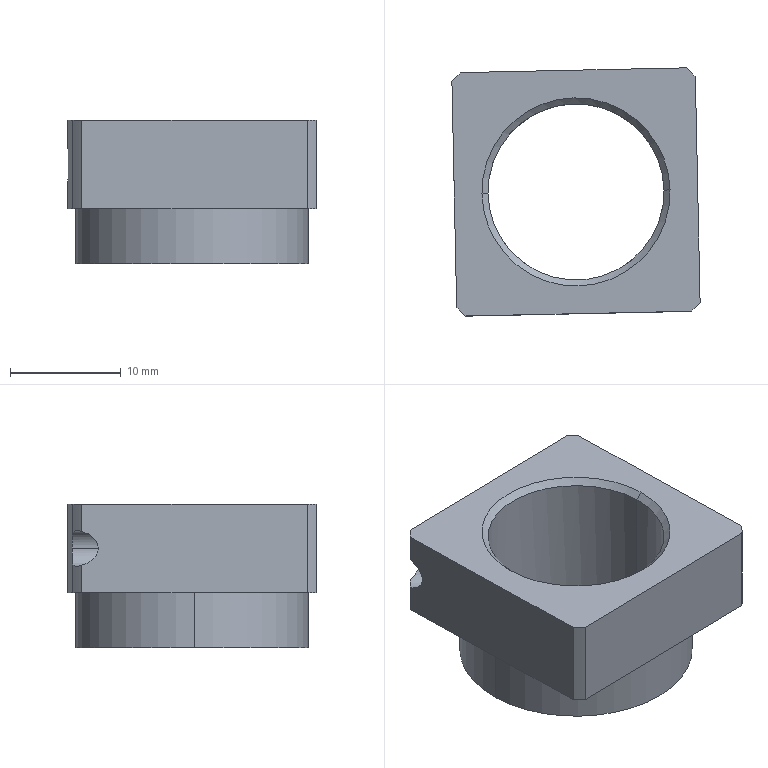Component | SolidWorks | CarrierBKE51-M17-1 | 1 solid | 22 faces | box 22.43 x 22.43 x 13 mm | volume 2936 mm3 | cylinder 11 | plane 7 | cone 4 | commonest cylinder face diameters 30 x5 15.917 x2 3.242 x2 21 x2
STEP:
#1=COLOUR_RGB('',0.7922,0.8196,0.9333);
#2=FILL_AREA_STYLE_COLOUR('',#1);
#3=FILL_AREA_STYLE('',(#2));
#4=SURFACE_STYLE_FILL_AREA(#3);
#5=SURFACE_SIDE_STYLE('',(#4));
#6=SURFACE_STYLE_USAGE(.BOTH.,#5);
#7=PRESENTATION_STYLE_ASSIGNMENT((#6));
#8=CARTESIAN_POINT('',(-0.5726,0.006608,1.081));
#9=VERTEX_POINT('',#8);
#10=CARTESIAN_POINT('',(-1.199,-0.006608,1.081));
#11=VERTEX_POINT('',#10);
#12=CARTESIAN_POINT('',(-0.8858,-0.,1.081));
#13=DIRECTION('',(0.,0.,-1.));
#14=DIRECTION('',(-0.9998,-0.02109,0.));
#15=AXIS2_PLACEMENT_3D('',#12,#13,#14);
#16=CIRCLE('',#15,0.3133);
#17=EDGE_CURVE('',#9,#11,#16,.T.);
#18=ORIENTED_EDGE('',*,*,#17,.F.);
#19=CARTESIAN_POINT('',(-0.5726,0.006608,0.6119));
#20=VERTEX_POINT('',#19);
#21=CARTESIAN_POINT('',(-0.5726,0.006608,1.102));
#22=DIRECTION('',(0.,0.,-1.));
#23=VECTOR('',#22,39.37);
#24=LINE('',#21,#23);
#25=EDGE_CURVE('',#9,#20,#24,.T.);
#26=ORIENTED_EDGE('',*,*,#25,.T.);
#27=CARTESIAN_POINT('',(-0.8792,-0.3133,0.6119));
#28=VERTEX_POINT('',#27);
#29=CARTESIAN_POINT('',(-0.8858,-0.,0.6119));
#30=DIRECTION('',(0.,0.,1.));
#31=DIRECTION('',(-0.9998,-0.02109,0.));
#32=AXIS2_PLACEMENT_3D('',#29,#30,#31);
#33=CIRCLE('',#32,0.3133);
#34=EDGE_CURVE('',#28,#20,#33,.T.);
#35=ORIENTED_EDGE('',*,*,#34,.F.);
#36=CARTESIAN_POINT('',(-1.199,-0.006608,0.6119));
#37=VERTEX_POINT('',#36);
#38=CARTESIAN_POINT('',(-0.8858,-0.,0.6119));
#39=DIRECTION('',(0.,0.,1.));
#40=DIRECTION('',(-0.9998,-0.02109,0.));
#41=AXIS2_PLACEMENT_3D('',#38,#39,#40);
#42=CIRCLE('',#41,0.3133);
#43=EDGE_CURVE('',#37,#28,#42,.T.);
#44=ORIENTED_EDGE('',*,*,#43,.F.);
#45=CARTESIAN_POINT('',(-1.199,-0.006608,1.102));
#46=DIRECTION('',(0.,0.,-1.));
#47=VECTOR('',#46,39.37);
#48=LINE('',#45,#47);
#49=EDGE_CURVE('',#11,#37,#48,.T.);
#50=ORIENTED_EDGE('',*,*,#49,.F.);
#51=EDGE_LOOP('',(#18,#26,#35,#44,#50));
#52=FACE_OUTER_BOUND('',#51,.T.);
#53=CARTESIAN_POINT('',(-0.8858,-0.,1.102));
#54=DIRECTION('',(0.,0.,-1.));
#55=DIRECTION('',(-0.9998,-0.02109,0.));
#56=AXIS2_PLACEMENT_3D('',#53,#54,#55);
#57=CYLINDRICAL_SURFACE('',#56,0.3133);
#58=ADVANCED_FACE('',(#52),#57,.F.);
#59=CARTESIAN_POINT('',(-1.063,0.2584,0.9449));
#60=VERTEX_POINT('',#59);
#61=CARTESIAN_POINT('',(-1.151,0.1662,0.9449));
#62=VERTEX_POINT('',#61);
#63=CARTESIAN_POINT('',(-1.063,0.2584,0.9449));
#64=CARTESIAN_POINT('',(-1.063,0.2584,0.9491));
#65=CARTESIAN_POINT('',(-1.063,0.2581,0.9533));
#66=CARTESIAN_POINT('',(-1.065,0.2572,0.9614));
#67=CARTESIAN_POINT('',(-1.066,0.2565,0.9655));
#68=CARTESIAN_POINT('',(-1.069,0.2546,0.9732));
#69=CARTESIAN_POINT('',(-1.07,0.2534,0.9769));
#70=CARTESIAN_POINT('',(-1.074,0.2506,0.9838));
#71=CARTESIAN_POINT('',(-1.076,0.249,0.9871));
#72=CARTESIAN_POINT('',(-1.083,0.2435,0.9959));
#73=CARTESIAN_POINT('',(-1.089,0.239,1.001));
#74=CARTESIAN_POINT('',(-1.1,0.2287,1.007));
#75=CARTESIAN_POINT('',(-1.106,0.2229,1.009));
#76=CARTESIAN_POINT('',(-1.115,0.2138,1.009));
#77=CARTESIAN_POINT('',(-1.118,0.2107,1.008));
#78=CARTESIAN_POINT('',(-1.123,0.2046,1.007));
#79=CARTESIAN_POINT('',(-1.126,0.2015,1.005));
#80=CARTESIAN_POINT('',(-1.133,0.1925,1.001));
#81=CARTESIAN_POINT('',(-1.137,0.1869,0.9959));
#82=CARTESIAN_POINT('',(-1.143,0.1796,0.9871));
#83=CARTESIAN_POINT('',(-1.144,0.1774,0.9838));
#84=CARTESIAN_POINT('',(-1.147,0.1735,0.9769));
#85=CARTESIAN_POINT('',(-1.148,0.1718,0.9732));
#86=CARTESIAN_POINT('',(-1.15,0.169,0.9655));
#87=CARTESIAN_POINT('',(-1.15,0.168,0.9615));
#88=CARTESIAN_POINT('',(-1.151,0.1666,0.9533));
#89=CARTESIAN_POINT('',(-1.151,0.1662,0.9491));
#90=CARTESIAN_POINT('',(-1.151,0.1662,0.9449));
#91=B_SPLINE_CURVE_WITH_KNOTS('',3,(#63,#64,#65,#66,#67,#68,#69,#70,#71,#72,#73,#74,#75,#76,#77,#78,#79,#80,#81,#82,#83,#84,#85,#86,#87,#88,#89,#90),.UNSPECIFIED.,.F.,.F.,(4,2,2,2,2,2,2,2,2,2,2,2,2,4),(0.004894,0.005212,0.005529,0.005847,0.006164,0.006799,0.007434,0.007752,0.008069,0.008704,0.009022,0.00934,0.009657,0.009975),.UNSPECIFIED.);
#92=EDGE_CURVE('',#60,#62,#91,.T.);
#93=ORIENTED_EDGE('',*,*,#92,.T.);
#94=CARTESIAN_POINT('',(-1.326,0.3336,0.9449));
#95=VERTEX_POINT('',#94);
#96=CARTESIAN_POINT('',(-1.143,0.1583,0.9449));
#97=DIRECTION('',(-0.7219,0.692,0.));
#98=VECTOR('',#97,39.37);
#99=LINE('',#96,#98);
#100=EDGE_CURVE('',#62,#95,#99,.T.);
#101=ORIENTED_EDGE('',*,*,#100,.T.);
#102=CARTESIAN_POINT('',(-1.327,0.3923,1.005));
#103=VERTEX_POINT('',#102);
#104=CARTESIAN_POINT('',(-1.327,0.3923,1.005));
#105=CARTESIAN_POINT('',(-1.326,0.3558,0.995));
#106=CARTESIAN_POINT('',(-1.326,0.3336,0.9724));
#107=CARTESIAN_POINT('',(-1.326,0.3336,0.9449));
#108=(BOUNDED_CURVE()B_SPLINE_CURVE(3,(#104,#105,#106,#107),.UNSPECIFIED.,.F.,.T.)B_SPLINE_CURVE_WITH_KNOTS((4,4),(1.928,3.142),.UNSPECIFIED.)CURVE()GEOMETRIC_REPRESENTATION_ITEM()RATIONAL_B_SPLINE_CURVE((1.,0.881,0.881,1.))REPRESENTATION_ITEM(''));
#109=EDGE_CURVE('',#103,#95,#108,.T.);
#110=ORIENTED_EDGE('',*,*,#109,.F.);
#111=CARTESIAN_POINT('',(-1.296,0.4245,1.005));
#112=VERTEX_POINT('',#111);
#113=CARTESIAN_POINT('',(-1.296,0.4245,1.005));
#114=CARTESIAN_POINT('',(-1.302,0.4195,1.007));
#115=CARTESIAN_POINT('',(-1.307,0.4142,1.009));
#116=CARTESIAN_POINT('',(-1.317,0.4032,1.009));
#117=CARTESIAN_POINT('',(-1.322,0.3976,1.007));
#118=CARTESIAN_POINT('',(-1.327,0.3923,1.005));
#119=B_SPLINE_CURVE_WITH_KNOTS('',3,(#113,#114,#115,#116,#117,#118),.UNSPECIFIED.,.F.,.F.,(4,2,4),(0.,0.0005764,0.001153),.UNSPECIFIED.);
#120=EDGE_CURVE('',#112,#103,#119,.T.);
#121=ORIENTED_EDGE('',*,*,#120,.F.);
#122=CARTESIAN_POINT('',(-1.238,0.4257,0.9449));
#123=VERTEX_POINT('',#122);
#124=CARTESIAN_POINT('',(-1.238,0.4257,0.9449));
#125=CARTESIAN_POINT('',(-1.238,0.4257,0.9724));
#126=CARTESIAN_POINT('',(-1.26,0.4253,0.995));
#127=CARTESIAN_POINT('',(-1.296,0.4245,1.005));
#128=(BOUNDED_CURVE()B_SPLINE_CURVE(3,(#124,#125,#126,#127),.UNSPECIFIED.,.F.,.F.)B_SPLINE_CURVE_WITH_KNOTS((4,4),(3.142,4.355),.UNSPECIFIED.)CURVE()GEOMETRIC_REPRESENTATION_ITEM()RATIONAL_B_SPLINE_CURVE((1.,0.881,0.881,1.))REPRESENTATION_ITEM(''));
#129=EDGE_CURVE('',#123,#112,#128,.T.);
#130=ORIENTED_EDGE('',*,*,#129,.F.);
#131=CARTESIAN_POINT('',(-1.055,0.2504,0.9449));
#132=DIRECTION('',(-0.7219,0.692,0.));
#133=VECTOR('',#132,39.37);
#134=LINE('',#131,#133);
#135=EDGE_CURVE('',#60,#123,#134,.T.);
#136=ORIENTED_EDGE('',*,*,#135,.F.);
#137=EDGE_LOOP('',(#93,#101,#110,#121,#130,#136));
#138=FACE_OUTER_BOUND('',#137,.T.);
#139=CARTESIAN_POINT('',(-1.099,0.2043,0.9449));
#140=DIRECTION('',(-0.7219,0.692,0.));
#141=DIRECTION('',(0.692,0.7219,0.));
#142=AXIS2_PLACEMENT_3D('',#139,#140,#141);
#143=CYLINDRICAL_SURFACE('',#142,0.06382);
#144=ADVANCED_FACE('',(#138),#143,.F.);
#145=ORIENTED_EDGE('',*,*,#34,.T.);
#146=CARTESIAN_POINT('',(-0.8924,0.3133,0.6119));
#147=VERTEX_POINT('',#146);
#148=CARTESIAN_POINT('',(-0.8858,-0.,0.6119));
#149=DIRECTION('',(0.,0.,1.));
#150=DIRECTION('',(-0.9998,-0.02109,0.));
#151=AXIS2_PLACEMENT_3D('',#148,#149,#150);
#152=CIRCLE('',#151,0.3133);
#153=EDGE_CURVE('',#20,#147,#152,.T.);
#154=ORIENTED_EDGE('',*,*,#153,.T.);
#155=CARTESIAN_POINT('',(-0.8929,0.3346,0.5906));
#156=VERTEX_POINT('',#155);
#157=CARTESIAN_POINT('',(-0.8929,0.3346,0.5906));
#158=DIRECTION('',(-0.01491,0.7069,-0.7071));
#159=VECTOR('',#158,39.37);
#160=LINE('',#157,#159);
#161=EDGE_CURVE('',#147,#156,#160,.T.);
#162=ORIENTED_EDGE('',*,*,#161,.T.);
#163=CARTESIAN_POINT('',(-0.8788,-0.3346,0.5906));
#164=VERTEX_POINT('',#163);
#165=CARTESIAN_POINT('',(-0.8858,-0.,0.5906));
#166=DIRECTION('',(0.,-0.,1.));
#167=DIRECTION('',(0.02109,-0.9998,0.));
#168=AXIS2_PLACEMENT_3D('',#165,#166,#167);
#169=CIRCLE('',#168,0.3346);
#170=EDGE_CURVE('',#164,#156,#169,.T.);
#171=ORIENTED_EDGE('',*,*,#170,.F.);
#172=CARTESIAN_POINT('',(-0.8788,-0.3346,0.5906));
#173=DIRECTION('',(0.01491,-0.7069,-0.7071));
#174=VECTOR('',#173,39.37);
#175=LINE('',#172,#174);
#176=EDGE_CURVE('',#28,#164,#175,.T.);
#177=ORIENTED_EDGE('',*,*,#176,.F.);
#178=EDGE_LOOP('',(#145,#154,#162,#171,#177));
#179=FACE_OUTER_BOUND('',#178,.T.);
#180=CARTESIAN_POINT('',(-0.8858,-0.,0.5906));
#181=DIRECTION('',(-0.,0.,-1.));
#182=DIRECTION('',(0.02109,-0.9998,0.));
#183=AXIS2_PLACEMENT_3D('',#180,#181,#182);
#184=CONICAL_SURFACE('',#183,0.3346,0.7854);
#185=ADVANCED_FACE('',(#179),#184,.F.);
#186=ORIENTED_EDGE('',*,*,#17,.T.);
#187=CARTESIAN_POINT('',(-1.22,-0.007058,1.102));
#188=VERTEX_POINT('',#187);
#189=CARTESIAN_POINT('',(-1.22,-0.007058,1.102));
#190=DIRECTION('',(-0.7069,-0.01491,0.7071));
#191=VECTOR('',#190,39.37);
#192=LINE('',#189,#191);
#193=EDGE_CURVE('',#11,#188,#192,.T.);
#194=ORIENTED_EDGE('',*,*,#193,.T.);
#195=CARTESIAN_POINT('',(-0.5513,0.007058,1.102));
#196=VERTEX_POINT('',#195);
#197=CARTESIAN_POINT('',(-0.8858,-0.,1.102));
#198=DIRECTION('',(0.,0.,-1.));
#199=DIRECTION('',(0.9998,0.02109,0.));
#200=AXIS2_PLACEMENT_3D('',#197,#198,#199);
#201=CIRCLE('',#200,0.3346);
#202=EDGE_CURVE('',#196,#188,#201,.T.);
#203=ORIENTED_EDGE('',*,*,#202,.F.);
#204=CARTESIAN_POINT('',(-0.5513,0.007058,1.102));
#205=DIRECTION('',(0.7069,0.01491,0.7071));
#206=VECTOR('',#205,39.37);
#207=LINE('',#204,#206);
#208=EDGE_CURVE('',#9,#196,#207,.T.);
#209=ORIENTED_EDGE('',*,*,#208,.F.);
#210=EDGE_LOOP('',(#186,#194,#203,#209));
#211=FACE_OUTER_BOUND('',#210,.T.);
#212=CARTESIAN_POINT('',(-0.8858,-0.,1.102));
#213=DIRECTION('',(0.,0.,1.));
#214=DIRECTION('',(0.9998,0.02109,0.));
#215=AXIS2_PLACEMENT_3D('',#212,#213,#214);
#216=CONICAL_SURFACE('',#215,0.3346,0.7854);
#217=ADVANCED_FACE('',(#211),#216,.F.);
#218=CARTESIAN_POINT('',(-0.4725,0.008718,0.7874));
#219=VERTEX_POINT('',#218);
#220=CARTESIAN_POINT('',(-1.299,-0.008718,0.7874));
#221=VERTEX_POINT('',#220);
#222=CARTESIAN_POINT('',(-0.8858,-0.,0.7874));
#223=DIRECTION('',(0.,0.,1.));
#224=DIRECTION('',(-0.9998,-0.02109,0.));
#225=AXIS2_PLACEMENT_3D('',#222,#223,#224);
#226=CIRCLE('',#225,0.4134);
#227=EDGE_CURVE('',#219,#221,#226,.T.);
#228=ORIENTED_EDGE('',*,*,#227,.F.);
#229=CARTESIAN_POINT('',(-0.4725,0.008718,0.5906));
#230=VERTEX_POINT('',#229);
#231=CARTESIAN_POINT('',(-0.4725,0.008718,0.5906));
#232=DIRECTION('',(0.,0.,-1.));
#233=VECTOR('',#232,39.37);
#234=LINE('',#231,#233);
#235=EDGE_CURVE('',#219,#230,#234,.T.);
#236=ORIENTED_EDGE('',*,*,#235,.T.);
#237=CARTESIAN_POINT('',(-1.299,-0.008718,0.5906));
#238=VERTEX_POINT('',#237);
#239=CARTESIAN_POINT('',(-0.8858,-0.,0.5906));
#240=DIRECTION('',(0.,0.,-1.));
#241=DIRECTION('',(-0.9998,-0.02109,0.));
#242=AXIS2_PLACEMENT_3D('',#239,#240,#241);
#243=CIRCLE('',#242,0.4134);
#244=EDGE_CURVE('',#238,#230,#243,.T.);
#245=ORIENTED_EDGE('',*,*,#244,.F.);
#246=CARTESIAN_POINT('',(-1.299,-0.008718,0.5906));
#247=DIRECTION('',(0.,0.,-1.));
#248=VECTOR('',#247,39.37);
#249=LINE('',#246,#248);
#250=EDGE_CURVE('',#221,#238,#249,.T.);
#251=ORIENTED_EDGE('',*,*,#250,.F.);
#252=EDGE_LOOP('',(#228,#236,#245,#251));
#253=FACE_OUTER_BOUND('',#252,.T.);
#254=CARTESIAN_POINT('',(-0.8858,-0.,0.5906));
#255=DIRECTION('',(0.,0.,-1.));
#256=DIRECTION('',(-0.9998,-0.02109,0.));
#257=AXIS2_PLACEMENT_3D('',#254,#255,#256);
#258=CYLINDRICAL_SURFACE('',#257,0.4134);
#259=ADVANCED_FACE('',(#253),#258,.T.);
#260=ORIENTED_EDGE('',*,*,#25,.F.);
#261=CARTESIAN_POINT('',(-0.8858,-0.,1.081));
#262=DIRECTION('',(0.,0.,-1.));
#263=DIRECTION('',(-0.9998,-0.02109,0.));
#264=AXIS2_PLACEMENT_3D('',#261,#262,#263);
#265=CIRCLE('',#264,0.3133);
#266=EDGE_CURVE('',#11,#9,#265,.T.);
#267=ORIENTED_EDGE('',*,*,#266,.F.);
#268=ORIENTED_EDGE('',*,*,#49,.T.);
#269=CARTESIAN_POINT('',(-0.8858,-0.,0.6119));
#270=DIRECTION('',(0.,0.,1.));
#271=DIRECTION('',(-0.9998,-0.02109,0.));
#272=AXIS2_PLACEMENT_3D('',#269,#270,#271);
#273=CIRCLE('',#272,0.3133);
#274=EDGE_CURVE('',#147,#37,#273,.T.);
#275=ORIENTED_EDGE('',*,*,#274,.F.);
#276=ORIENTED_EDGE('',*,*,#153,.F.);
#277=EDGE_LOOP('',(#260,#267,#268,#275,#276));
#278=FACE_OUTER_BOUND('',#277,.T.);
#279=ORIENTED_EDGE('',*,*,#92,.F.);
#280=CARTESIAN_POINT('',(-1.151,0.1662,0.9449));
#281=CARTESIAN_POINT('',(-1.151,0.1662,0.9407));
#282=CARTESIAN_POINT('',(-1.151,0.1666,0.9365));
#283=CARTESIAN_POINT('',(-1.15,0.168,0.9283));
#284=CARTESIAN_POINT('',(-1.15,0.169,0.9243));
#285=CARTESIAN_POINT('',(-1.148,0.1718,0.9165));
#286=CARTESIAN_POINT('',(-1.147,0.1735,0.9128));
#287=CARTESIAN_POINT('',(-1.144,0.1774,0.9059));
#288=CARTESIAN_POINT('',(-1.143,0.1796,0.9027));
#289=CARTESIAN_POINT('',(-1.139,0.1845,0.8968));
#290=CARTESIAN_POINT('',(-1.137,0.1871,0.8941));
#291=CARTESIAN_POINT('',(-1.133,0.1926,0.8895));
#292=CARTESIAN_POINT('',(-1.131,0.1955,0.8875));
#293=CARTESIAN_POINT('',(-1.126,0.2015,0.8843));
#294=CARTESIAN_POINT('',(-1.123,0.2046,0.8831));
#295=CARTESIAN_POINT('',(-1.118,0.2107,0.8815));
#296=CARTESIAN_POINT('',(-1.115,0.2138,0.8811));
#297=CARTESIAN_POINT('',(-1.106,0.2229,0.8811));
#298=CARTESIAN_POINT('',(-1.1,0.2287,0.8828));
#299=CARTESIAN_POINT('',(-1.089,0.239,0.8891));
#300=CARTESIAN_POINT('',(-1.083,0.2435,0.8939));
#301=CARTESIAN_POINT('',(-1.076,0.249,0.9027));
#302=CARTESIAN_POINT('',(-1.074,0.2506,0.906));
#303=CARTESIAN_POINT('',(-1.07,0.2534,0.9129));
#304=CARTESIAN_POINT('',(-1.069,0.2546,0.9165));
#305=CARTESIAN_POINT('',(-1.066,0.2565,0.9243));
#306=CARTESIAN_POINT('',(-1.065,0.2572,0.9283));
#307=CARTESIAN_POINT('',(-1.063,0.2581,0.9365));
#308=CARTESIAN_POINT('',(-1.063,0.2584,0.9407));
#309=CARTESIAN_POINT('',(-1.063,0.2584,0.9449));
#310=B_SPLINE_CURVE_WITH_KNOTS('',3,(#280,#281,#282,#283,#284,#285,#286,#287,#288,#289,#290,#291,#292,#293,#294,#295,#296,#297,#298,#299,#300,#301,#302,#303,#304,#305,#306,#307,#308,#309),.UNSPECIFIED.,.F.,.F.,(4,2,2,2,2,2,2,2,2,2,2,2,2,2,4),(0.009975,0.01029,0.01061,0.01093,0.01124,0.01156,0.01188,0.0122,0.01251,0.01315,0.01378,0.0141,0.01442,0.01474,0.01506),.UNSPECIFIED.);
#311=EDGE_CURVE('',#62,#60,#310,.T.);
#312=ORIENTED_EDGE('',*,*,#311,.F.);
#313=EDGE_LOOP('',(#279,#312));
#314=FACE_BOUND('',#313,.T.);
#315=CARTESIAN_POINT('',(-0.8858,-0.,1.102));
#316=DIRECTION('',(0.,0.,-1.));
#317=DIRECTION('',(-0.9998,-0.02109,0.));
#318=AXIS2_PLACEMENT_3D('',#315,#316,#317);
#319=CYLINDRICAL_SURFACE('',#318,0.3133);
#320=ADVANCED_FACE('',(#278,#314),#319,.F.);
#321=ORIENTED_EDGE('',*,*,#100,.F.);
#322=ORIENTED_EDGE('',*,*,#311,.T.);
#323=ORIENTED_EDGE('',*,*,#135,.T.);
#324=CARTESIAN_POINT('',(-1.296,0.4245,0.8851));
#325=VERTEX_POINT('',#324);
#326=CARTESIAN_POINT('',(-1.296,0.4245,0.8851));
#327=CARTESIAN_POINT('',(-1.26,0.4253,0.8947));
#328=CARTESIAN_POINT('',(-1.238,0.4257,0.9173));
#329=CARTESIAN_POINT('',(-1.238,0.4257,0.9449));
#330=(BOUNDED_CURVE()B_SPLINE_CURVE(3,(#326,#327,#328,#329),.UNSPECIFIED.,.F.,.T.)B_SPLINE_CURVE_WITH_KNOTS((4,4),(1.928,3.142),.UNSPECIFIED.)CURVE()GEOMETRIC_REPRESENTATION_ITEM()RATIONAL_B_SPLINE_CURVE((1.,0.881,0.881,1.))REPRESENTATION_ITEM(''));
#331=EDGE_CURVE('',#325,#123,#330,.T.);
#332=ORIENTED_EDGE('',*,*,#331,.F.);
#333=CARTESIAN_POINT('',(-1.327,0.3923,0.8851));
#334=VERTEX_POINT('',#333);
#335=CARTESIAN_POINT('',(-1.327,0.3923,0.8851));
#336=CARTESIAN_POINT('',(-1.322,0.3976,0.8824));
#337=CARTESIAN_POINT('',(-1.317,0.4032,0.8811));
#338=CARTESIAN_POINT('',(-1.307,0.4142,0.8811));
#339=CARTESIAN_POINT('',(-1.302,0.4195,0.8824));
#340=CARTESIAN_POINT('',(-1.296,0.4245,0.8851));
#341=B_SPLINE_CURVE_WITH_KNOTS('',3,(#335,#336,#337,#338,#339,#340),.UNSPECIFIED.,.F.,.F.,(4,2,4),(0.,0.0005764,0.001153),.UNSPECIFIED.);
#342=EDGE_CURVE('',#334,#325,#341,.T.);
#343=ORIENTED_EDGE('',*,*,#342,.F.);
#344=CARTESIAN_POINT('',(-1.326,0.3336,0.9449));
#345=CARTESIAN_POINT('',(-1.326,0.3336,0.9173));
#346=CARTESIAN_POINT('',(-1.326,0.3558,0.8947));
#347=CARTESIAN_POINT('',(-1.327,0.3923,0.8851));
#348=(BOUNDED_CURVE()B_SPLINE_CURVE(3,(#344,#345,#346,#347),.UNSPECIFIED.,.F.,.F.)B_SPLINE_CURVE_WITH_KNOTS((4,4),(3.142,4.355),.UNSPECIFIED.)CURVE()GEOMETRIC_REPRESENTATION_ITEM()RATIONAL_B_SPLINE_CURVE((1.,0.881,0.881,1.))REPRESENTATION_ITEM(''));
#349=EDGE_CURVE('',#95,#334,#348,.T.);
#350=ORIENTED_EDGE('',*,*,#349,.F.);
#351=EDGE_LOOP('',(#321,#322,#323,#332,#343,#350));
#352=FACE_OUTER_BOUND('',#351,.T.);
#353=CARTESIAN_POINT('',(-1.099,0.2043,0.9449));
#354=DIRECTION('',(-0.7219,0.692,0.));
#355=DIRECTION('',(0.692,0.7219,0.));
#356=AXIS2_PLACEMENT_3D('',#353,#354,#355);
#357=CYLINDRICAL_SURFACE('',#356,0.06382);
#358=ADVANCED_FACE('',(#352),#357,.F.);
#359=ORIENTED_EDGE('',*,*,#161,.F.);
#360=ORIENTED_EDGE('',*,*,#274,.T.);
#361=ORIENTED_EDGE('',*,*,#43,.T.);
#362=ORIENTED_EDGE('',*,*,#176,.T.);
#363=CARTESIAN_POINT('',(-0.8858,-0.,0.5906));
#364=DIRECTION('',(0.,-0.,1.));
#365=DIRECTION('',(0.02109,-0.9998,0.));
#366=AXIS2_PLACEMENT_3D('',#363,#364,#365);
#367=CIRCLE('',#366,0.3346);
#368=EDGE_CURVE('',#156,#164,#367,.T.);
#369=ORIENTED_EDGE('',*,*,#368,.F.);
#370=EDGE_LOOP('',(#359,#360,#361,#362,#369));
#371=FACE_OUTER_BOUND('',#370,.T.);
#372=CARTESIAN_POINT('',(-0.8858,-0.,0.5906));
#373=DIRECTION('',(-0.,0.,-1.));
#374=DIRECTION('',(0.02109,-0.9998,0.));
#375=AXIS2_PLACEMENT_3D('',#372,#373,#374);
#376=CONICAL_SURFACE('',#375,0.3346,0.7854);
#377=ADVANCED_FACE('',(#371),#376,.F.);
#378=ORIENTED_EDGE('',*,*,#193,.F.);
#379=ORIENTED_EDGE('',*,*,#266,.T.);
#380=ORIENTED_EDGE('',*,*,#208,.T.);
#381=CARTESIAN_POINT('',(-0.8858,-0.,1.102));
#382=DIRECTION('',(0.,0.,-1.));
#383=DIRECTION('',(0.9998,0.02109,0.));
#384=AXIS2_PLACEMENT_3D('',#381,#382,#383);
#385=CIRCLE('',#384,0.3346);
#386=EDGE_CURVE('',#188,#196,#385,.T.);
#387=ORIENTED_EDGE('',*,*,#386,.F.);
#388=EDGE_LOOP('',(#378,#379,#380,#387));
#389=FACE_OUTER_BOUND('',#388,.T.);
#390=CARTESIAN_POINT('',(-0.8858,-0.,1.102));
#391=DIRECTION('',(0.,0.,1.));
#392=DIRECTION('',(0.9998,0.02109,0.));
#393=AXIS2_PLACEMENT_3D('',#390,#391,#392);
#394=CONICAL_SURFACE('',#393,0.3346,0.7854);
#395=ADVANCED_FACE('',(#389),#394,.F.);
#396=ORIENTED_EDGE('',*,*,#109,.T.);
#397=ORIENTED_EDGE('',*,*,#349,.T.);
#398=CARTESIAN_POINT('',(-1.327,0.3923,0.7874));
#399=VERTEX_POINT('',#398);
#400=CARTESIAN_POINT('',(-1.327,0.3923,0.7874));
#401=DIRECTION('',(0.,0.,1.));
#402=VECTOR('',#401,39.37);
#403=LINE('',#400,#402);
#404=EDGE_CURVE('',#399,#334,#403,.T.);
#405=ORIENTED_EDGE('',*,*,#404,.F.);
#406=CARTESIAN_POINT('',(-1.31,-0.4105,0.7874));
#407=VERTEX_POINT('',#406);
#408=CARTESIAN_POINT('',(-1.31,-0.4105,0.7874));
#409=DIRECTION('',(-0.02109,0.9998,0.));
#410=VECTOR('',#409,39.37);
#411=LINE('',#408,#410);
#412=EDGE_CURVE('',#407,#399,#411,.T.);
#413=ORIENTED_EDGE('',*,*,#412,.F.);
#414=CARTESIAN_POINT('',(-1.31,-0.4105,1.102));
#415=VERTEX_POINT('',#414);
#416=CARTESIAN_POINT('',(-1.31,-0.4105,0.7874));
#417=DIRECTION('',(0.,0.,-1.));
#418=VECTOR('',#417,39.37);
#419=LINE('',#416,#418);
#420=EDGE_CURVE('',#415,#407,#419,.T.);
#421=ORIENTED_EDGE('',*,*,#420,.F.);
#422=CARTESIAN_POINT('',(-1.327,0.3923,1.102));
#423=VERTEX_POINT('',#422);
#424=CARTESIAN_POINT('',(-1.31,-0.4105,1.102));
#425=DIRECTION('',(0.02109,-0.9998,0.));
#426=VECTOR('',#425,39.37);
#427=LINE('',#424,#426);
#428=EDGE_CURVE('',#423,#415,#427,.T.);
#429=ORIENTED_EDGE('',*,*,#428,.F.);
#430=CARTESIAN_POINT('',(-1.327,0.3923,0.7874));
#431=DIRECTION('',(0.,0.,1.));
#432=VECTOR('',#431,39.37);
#433=LINE('',#430,#432);
#434=EDGE_CURVE('',#103,#423,#433,.T.);
#435=ORIENTED_EDGE('',*,*,#434,.F.);
#436=EDGE_LOOP('',(#396,#397,#405,#413,#421,#429,#435));
#437=FACE_OUTER_BOUND('',#436,.T.);
#438=CARTESIAN_POINT('',(-1.31,-0.4105,0.7874));
#439=DIRECTION('',(0.9998,0.02109,0.));
#440=DIRECTION('',(0.,0.,-1.));
#441=AXIS2_PLACEMENT_3D('',#438,#439,#440);
#442=PLANE('',#441);
#443=ADVANCED_FACE('',(#437),#442,.F.);
#444=CARTESIAN_POINT('',(-1.296,0.4245,1.102));
#445=VERTEX_POINT('',#444);
#446=CARTESIAN_POINT('',(-1.296,0.4245,0.7874));
#447=DIRECTION('',(0.,0.,-1.));
#448=VECTOR('',#447,39.37);
#449=LINE('',#446,#448);
#450=EDGE_CURVE('',#445,#112,#449,.T.);
#451=ORIENTED_EDGE('',*,*,#450,.F.);
#452=CARTESIAN_POINT('',(-0.4936,0.4414,1.102));
#453=VERTEX_POINT('',#452);
#454=CARTESIAN_POINT('',(-1.296,0.4245,1.102));
#455=DIRECTION('',(-0.9998,-0.02109,0.));
#456=VECTOR('',#455,39.37);
#457=LINE('',#454,#456);
#458=EDGE_CURVE('',#453,#445,#457,.T.);
#459=ORIENTED_EDGE('',*,*,#458,.F.);
#460=CARTESIAN_POINT('',(-0.4936,0.4414,0.7874));
#461=VERTEX_POINT('',#460);
#462=CARTESIAN_POINT('',(-0.4936,0.4414,0.7874));
#463=DIRECTION('',(0.,0.,1.));
#464=VECTOR('',#463,39.37);
#465=LINE('',#462,#464);
#466=EDGE_CURVE('',#461,#453,#465,.T.);
#467=ORIENTED_EDGE('',*,*,#466,.F.);
#468=CARTESIAN_POINT('',(-1.296,0.4245,0.7874));
#469=VERTEX_POINT('',#468);
#470=CARTESIAN_POINT('',(-1.296,0.4245,0.7874));
#471=DIRECTION('',(0.9998,0.02109,0.));
#472=VECTOR('',#471,39.37);
#473=LINE('',#470,#472);
#474=EDGE_CURVE('',#469,#461,#473,.T.);
#475=ORIENTED_EDGE('',*,*,#474,.F.);
#476=CARTESIAN_POINT('',(-1.296,0.4245,0.7874));
#477=DIRECTION('',(0.,0.,-1.));
#478=VECTOR('',#477,39.37);
#479=LINE('',#476,#478);
#480=EDGE_CURVE('',#325,#469,#479,.T.);
#481=ORIENTED_EDGE('',*,*,#480,.F.);
#482=ORIENTED_EDGE('',*,*,#331,.T.);
#483=ORIENTED_EDGE('',*,*,#129,.T.);
#484=EDGE_LOOP('',(#451,#459,#467,#475,#481,#482,#483));
#485=FACE_OUTER_BOUND('',#484,.T.);
#486=CARTESIAN_POINT('',(-1.296,0.4245,0.7874));
#487=DIRECTION('',(0.02109,-0.9998,0.));
#488=DIRECTION('',(0.,0.,1.));
#489=AXIS2_PLACEMENT_3D('',#486,#487,#488);
#490=PLANE('',#489);
#491=ADVANCED_FACE('',(#485),#490,.F.);
#492=ORIENTED_EDGE('',*,*,#170,.T.);
#493=ORIENTED_EDGE('',*,*,#368,.T.);
#494=EDGE_LOOP('',(#492,#493));
#495=FACE_BOUND('',#494,.T.);
#496=ORIENTED_EDGE('',*,*,#244,.T.);
#497=CARTESIAN_POINT('',(-0.8858,-0.,0.5906));
#498=DIRECTION('',(0.,0.,-1.));
#499=DIRECTION('',(-0.9998,-0.02109,0.));
#500=AXIS2_PLACEMENT_3D('',#497,#498,#499);
#501=CIRCLE('',#500,0.4134);
#502=EDGE_CURVE('',#230,#238,#501,.T.);
#503=ORIENTED_EDGE('',*,*,#502,.T.);
#504=EDGE_LOOP('',(#496,#503));
#505=FACE_OUTER_BOUND('',#504,.T.);
#506=CARTESIAN_POINT('',(-0.8858,-0.,0.5906));
#507=DIRECTION('',(0.,0.,-1.));
#508=DIRECTION('',(-0.9998,-0.02109,0.));
#509=AXIS2_PLACEMENT_3D('',#506,#507,#508);
#510=PLANE('',#509);
#511=ADVANCED_FACE('',(#495,#505),#510,.T.);
#512=ORIENTED_EDGE('',*,*,#202,.T.);
#513=ORIENTED_EDGE('',*,*,#386,.T.);
#514=EDGE_LOOP('',(#512,#513));
#515=FACE_BOUND('',#514,.T.);
#516=CARTESIAN_POINT('',(-0.4613,0.4105,1.102));
#517=VERTEX_POINT('',#516);
#518=CARTESIAN_POINT('',(-0.8858,0.,1.102));
#519=DIRECTION('',(0.,0.,-1.));
#520=DIRECTION('',(-0.9998,-0.02109,0.));
#521=AXIS2_PLACEMENT_3D('',#518,#519,#520);
#522=CIRCLE('',#521,0.5906);
#523=EDGE_CURVE('',#453,#517,#522,.T.);
#524=ORIENTED_EDGE('',*,*,#523,.F.);
#525=ORIENTED_EDGE('',*,*,#458,.T.);
#526=CARTESIAN_POINT('',(-0.8858,0.,1.102));
#527=DIRECTION('',(0.,0.,-1.));
#528=DIRECTION('',(-0.9998,-0.02109,0.));
#529=AXIS2_PLACEMENT_3D('',#526,#527,#528);
#530=CIRCLE('',#529,0.5906);
#531=EDGE_CURVE('',#423,#445,#530,.T.);
#532=ORIENTED_EDGE('',*,*,#531,.F.);
#533=ORIENTED_EDGE('',*,*,#428,.T.);
#534=CARTESIAN_POINT('',(-1.278,-0.4414,1.102));
#535=VERTEX_POINT('',#534);
#536=CARTESIAN_POINT('',(-0.8858,-0.,1.102));
#537=DIRECTION('',(0.,0.,-1.));
#538=DIRECTION('',(-0.9998,-0.02109,0.));
#539=AXIS2_PLACEMENT_3D('',#536,#537,#538);
#540=CIRCLE('',#539,0.5906);
#541=EDGE_CURVE('',#535,#415,#540,.T.);
#542=ORIENTED_EDGE('',*,*,#541,.F.);
#543=CARTESIAN_POINT('',(-0.4753,-0.4245,1.102));
#544=VERTEX_POINT('',#543);
#545=CARTESIAN_POINT('',(-0.8767,-0.433,1.102));
#546=DIRECTION('',(-0.9998,-0.02109,0.));
#547=VECTOR('',#546,39.37);
#548=LINE('',#545,#547);
#549=EDGE_CURVE('',#544,#535,#548,.T.);
#550=ORIENTED_EDGE('',*,*,#549,.F.);
#551=CARTESIAN_POINT('',(-0.4444,-0.3923,1.102));
#552=VERTEX_POINT('',#551);
#553=CARTESIAN_POINT('',(-0.8858,-0.,1.102));
#554=DIRECTION('',(0.,0.,-1.));
#555=DIRECTION('',(-0.9998,-0.02109,0.));
#556=AXIS2_PLACEMENT_3D('',#553,#554,#555);
#557=CIRCLE('',#556,0.5906);
#558=EDGE_CURVE('',#552,#544,#557,.T.);
#559=ORIENTED_EDGE('',*,*,#558,.F.);
#560=CARTESIAN_POINT('',(-0.4529,0.009133,1.102));
#561=DIRECTION('',(0.02109,-0.9998,0.));
#562=VECTOR('',#561,39.37);
#563=LINE('',#560,#562);
#564=EDGE_CURVE('',#517,#552,#563,.T.);
#565=ORIENTED_EDGE('',*,*,#564,.F.);
#566=EDGE_LOOP('',(#524,#525,#532,#533,#542,#550,#559,#565));
#567=FACE_OUTER_BOUND('',#566,.T.);
#568=CARTESIAN_POINT('',(-0.8858,-0.,1.102));
#569=DIRECTION('',(0.,0.,-1.));
#570=DIRECTION('',(-0.9998,-0.02109,0.));
#571=AXIS2_PLACEMENT_3D('',#568,#569,#570);
#572=PLANE('',#571);
#573=ADVANCED_FACE('',(#515,#567),#572,.F.);
#574=ORIENTED_EDGE('',*,*,#531,.T.);
#575=ORIENTED_EDGE('',*,*,#450,.T.);
#576=ORIENTED_EDGE('',*,*,#120,.T.);
#577=ORIENTED_EDGE('',*,*,#434,.T.);
#578=EDGE_LOOP('',(#574,#575,#576,#577));
#579=FACE_OUTER_BOUND('',#578,.T.);
#580=CARTESIAN_POINT('',(-0.8858,0.,0.7874));
#581=DIRECTION('',(0.,0.,-1.));
#582=DIRECTION('',(-0.9998,-0.02109,0.));
#583=AXIS2_PLACEMENT_3D('',#580,#581,#582);
#584=CYLINDRICAL_SURFACE('',#583,0.5906);
#585=ADVANCED_FACE('',(#579),#584,.T.);
#586=CARTESIAN_POINT('',(-0.8858,0.,0.7874));
#587=DIRECTION('',(0.,0.,1.));
#588=DIRECTION('',(-0.9998,-0.02109,0.));
#589=AXIS2_PLACEMENT_3D('',#586,#587,#588);
#590=CIRCLE('',#589,0.5906);
#591=EDGE_CURVE('',#469,#399,#590,.T.);
#592=ORIENTED_EDGE('',*,*,#591,.T.);
#593=ORIENTED_EDGE('',*,*,#404,.T.);
#594=ORIENTED_EDGE('',*,*,#342,.T.);
#595=ORIENTED_EDGE('',*,*,#480,.T.);
#596=EDGE_LOOP('',(#592,#593,#594,#595));
#597=FACE_OUTER_BOUND('',#596,.T.);
#598=CARTESIAN_POINT('',(-0.8858,0.,0.7874));
#599=DIRECTION('',(0.,0.,-1.));
#600=DIRECTION('',(-0.9998,-0.02109,0.));
#601=AXIS2_PLACEMENT_3D('',#598,#599,#600);
#602=CYLINDRICAL_SURFACE('',#601,0.5906);
#603=ADVANCED_FACE('',(#597),#602,.T.);
#604=CARTESIAN_POINT('',(-0.8858,-0.,0.7874));
#605=DIRECTION('',(0.,0.,1.));
#606=DIRECTION('',(-0.9998,-0.02109,0.));
#607=AXIS2_PLACEMENT_3D('',#604,#605,#606);
#608=CIRCLE('',#607,0.4134);
#609=EDGE_CURVE('',#221,#219,#608,.T.);
#610=ORIENTED_EDGE('',*,*,#609,.T.);
#611=ORIENTED_EDGE('',*,*,#227,.T.);
#612=EDGE_LOOP('',(#610,#611));
#613=FACE_BOUND('',#612,.T.);
#614=ORIENTED_EDGE('',*,*,#474,.T.);
#615=CARTESIAN_POINT('',(-0.4613,0.4105,0.7874));
#616=VERTEX_POINT('',#615);
#617=CARTESIAN_POINT('',(-0.8858,0.,0.7874));
#618=DIRECTION('',(0.,0.,-1.));
#619=DIRECTION('',(-0.9998,-0.02109,0.));
#620=AXIS2_PLACEMENT_3D('',#617,#618,#619);
#621=CIRCLE('',#620,0.5906);
#622=EDGE_CURVE('',#461,#616,#621,.T.);
#623=ORIENTED_EDGE('',*,*,#622,.T.);
#624=CARTESIAN_POINT('',(-0.4444,-0.3923,0.7874));
#625=VERTEX_POINT('',#624);
#626=CARTESIAN_POINT('',(-0.4529,0.009133,0.7874));
#627=DIRECTION('',(0.02109,-0.9998,0.));
#628=VECTOR('',#627,39.37);
#629=LINE('',#626,#628);
#630=EDGE_CURVE('',#616,#625,#629,.T.);
#631=ORIENTED_EDGE('',*,*,#630,.T.);
#632=CARTESIAN_POINT('',(-0.4753,-0.4245,0.7874));
#633=VERTEX_POINT('',#632);
#634=CARTESIAN_POINT('',(-0.8858,-0.,0.7874));
#635=DIRECTION('',(0.,0.,1.));
#636=DIRECTION('',(-0.9998,-0.02109,0.));
#637=AXIS2_PLACEMENT_3D('',#634,#635,#636);
#638=CIRCLE('',#637,0.5906);
#639=EDGE_CURVE('',#633,#625,#638,.T.);
#640=ORIENTED_EDGE('',*,*,#639,.F.);
#641=CARTESIAN_POINT('',(-1.278,-0.4414,0.7874));
#642=VERTEX_POINT('',#641);
#643=CARTESIAN_POINT('',(-0.8767,-0.433,0.7874));
#644=DIRECTION('',(-0.9998,-0.02109,0.));
#645=VECTOR('',#644,39.37);
#646=LINE('',#643,#645);
#647=EDGE_CURVE('',#633,#642,#646,.T.);
#648=ORIENTED_EDGE('',*,*,#647,.T.);
#649=CARTESIAN_POINT('',(-0.8858,-0.,0.7874));
#650=DIRECTION('',(0.,0.,-1.));
#651=DIRECTION('',(-0.9998,-0.02109,0.));
#652=AXIS2_PLACEMENT_3D('',#649,#650,#651);
#653=CIRCLE('',#652,0.5906);
#654=EDGE_CURVE('',#642,#407,#653,.T.);
#655=ORIENTED_EDGE('',*,*,#654,.T.);
#656=ORIENTED_EDGE('',*,*,#412,.T.);
#657=ORIENTED_EDGE('',*,*,#591,.F.);
#658=EDGE_LOOP('',(#614,#623,#631,#640,#648,#655,#656,#657));
#659=FACE_OUTER_BOUND('',#658,.T.);
#660=CARTESIAN_POINT('',(-0.8858,-0.,0.7874));
#661=DIRECTION('',(0.,0.,-1.));
#662=DIRECTION('',(-0.9998,-0.02109,0.));
#663=AXIS2_PLACEMENT_3D('',#660,#661,#662);
#664=PLANE('',#663);
#665=ADVANCED_FACE('',(#613,#659),#664,.T.);
#666=ORIENTED_EDGE('',*,*,#654,.F.);
#667=CARTESIAN_POINT('',(-1.278,-0.4414,0.7874));
#668=DIRECTION('',(0.,0.,1.));
#669=VECTOR('',#668,39.37);
#670=LINE('',#667,#669);
#671=EDGE_CURVE('',#642,#535,#670,.T.);
#672=ORIENTED_EDGE('',*,*,#671,.T.);
#673=ORIENTED_EDGE('',*,*,#541,.T.);
#674=ORIENTED_EDGE('',*,*,#420,.T.);
#675=EDGE_LOOP('',(#666,#672,#673,#674));
#676=FACE_OUTER_BOUND('',#675,.T.);
#677=CARTESIAN_POINT('',(-0.8858,-0.,0.7874));
#678=DIRECTION('',(0.,0.,-1.));
#679=DIRECTION('',(-0.9998,-0.02109,0.));
#680=AXIS2_PLACEMENT_3D('',#677,#678,#679);
#681=CYLINDRICAL_SURFACE('',#680,0.5906);
#682=ADVANCED_FACE('',(#676),#681,.T.);
#683=ORIENTED_EDGE('',*,*,#622,.F.);
#684=ORIENTED_EDGE('',*,*,#466,.T.);
#685=ORIENTED_EDGE('',*,*,#523,.T.);
#686=CARTESIAN_POINT('',(-0.4613,0.4105,0.7874));
#687=DIRECTION('',(0.,0.,-1.));
#688=VECTOR('',#687,39.37);
#689=LINE('',#686,#688);
#690=EDGE_CURVE('',#517,#616,#689,.T.);
#691=ORIENTED_EDGE('',*,*,#690,.T.);
#692=EDGE_LOOP('',(#683,#684,#685,#691));
#693=FACE_OUTER_BOUND('',#692,.T.);
#694=CARTESIAN_POINT('',(-0.8858,0.,0.7874));
#695=DIRECTION('',(0.,0.,-1.));
#696=DIRECTION('',(-0.9998,-0.02109,0.));
#697=AXIS2_PLACEMENT_3D('',#694,#695,#696);
#698=CYLINDRICAL_SURFACE('',#697,0.5906);
#699=ADVANCED_FACE('',(#693),#698,.T.);
#700=ORIENTED_EDGE('',*,*,#235,.F.);
#701=ORIENTED_EDGE('',*,*,#609,.F.);
#702=ORIENTED_EDGE('',*,*,#250,.T.);
#703=ORIENTED_EDGE('',*,*,#502,.F.);
#704=EDGE_LOOP('',(#700,#701,#702,#703));
#705=FACE_OUTER_BOUND('',#704,.T.);
#706=CARTESIAN_POINT('',(-0.8858,-0.,0.5906));
#707=DIRECTION('',(0.,0.,-1.));
#708=DIRECTION('',(-0.9998,-0.02109,0.));
#709=AXIS2_PLACEMENT_3D('',#706,#707,#708);
#710=CYLINDRICAL_SURFACE('',#709,0.4134);
#711=ADVANCED_FACE('',(#705),#710,.T.);
#712=CARTESIAN_POINT('',(-0.4444,-0.3923,0.7874));
#713=DIRECTION('',(0.,0.,1.));
#714=VECTOR('',#713,39.37);
#715=LINE('',#712,#714);
#716=EDGE_CURVE('',#625,#552,#715,.T.);
#717=ORIENTED_EDGE('',*,*,#716,.F.);
#718=ORIENTED_EDGE('',*,*,#630,.F.);
#719=ORIENTED_EDGE('',*,*,#690,.F.);
#720=ORIENTED_EDGE('',*,*,#564,.T.);
#721=EDGE_LOOP('',(#717,#718,#719,#720));
#722=FACE_OUTER_BOUND('',#721,.T.);
#723=CARTESIAN_POINT('',(-0.4613,0.4105,0.7874));
#724=DIRECTION('',(-0.9998,-0.02109,0.));
#725=DIRECTION('',(0.,0.,1.));
#726=AXIS2_PLACEMENT_3D('',#723,#724,#725);
#727=PLANE('',#726);
#728=ADVANCED_FACE('',(#722),#727,.F.);
#729=ORIENTED_EDGE('',*,*,#671,.F.);
#730=ORIENTED_EDGE('',*,*,#647,.F.);
#731=CARTESIAN_POINT('',(-0.4753,-0.4245,0.7874));
#732=DIRECTION('',(0.,0.,-1.));
#733=VECTOR('',#732,39.37);
#734=LINE('',#731,#733);
#735=EDGE_CURVE('',#544,#633,#734,.T.);
#736=ORIENTED_EDGE('',*,*,#735,.F.);
#737=ORIENTED_EDGE('',*,*,#549,.T.);
#738=EDGE_LOOP('',(#729,#730,#736,#737));
#739=FACE_OUTER_BOUND('',#738,.T.);
#740=CARTESIAN_POINT('',(-0.4753,-0.4245,0.7874));
#741=DIRECTION('',(-0.02109,0.9998,0.));
#742=DIRECTION('',(0.,0.,-1.));
#743=AXIS2_PLACEMENT_3D('',#740,#741,#742);
#744=PLANE('',#743);
#745=ADVANCED_FACE('',(#739),#744,.F.);
#746=ORIENTED_EDGE('',*,*,#639,.T.);
#747=ORIENTED_EDGE('',*,*,#716,.T.);
#748=ORIENTED_EDGE('',*,*,#558,.T.);
#749=ORIENTED_EDGE('',*,*,#735,.T.);
#750=EDGE_LOOP('',(#746,#747,#748,#749));
#751=FACE_OUTER_BOUND('',#750,.T.);
#752=CARTESIAN_POINT('',(-0.8858,-0.,0.7874));
#753=DIRECTION('',(0.,0.,-1.));
#754=DIRECTION('',(-0.9998,-0.02109,0.));
#755=AXIS2_PLACEMENT_3D('',#752,#753,#754);
#756=CYLINDRICAL_SURFACE('',#755,0.5906);
#757=ADVANCED_FACE('',(#751),#756,.T.);
#758=CLOSED_SHELL('',(#58,#144,#185,#217,#259,#320,#358,#377,#395,#443,#491,#511,#573,#585,#603,#665,#682,#699,#711,#728,#745,#757));
#759=MANIFOLD_SOLID_BREP('',#758);
#760=STYLED_ITEM('',(#7),#759);
#761=PRESENTATION_LAYER_ASSIGNMENT('','',(#760));
#762=CARTESIAN_POINT('',(0.,0.,0.));
#763=DIRECTION('',(0.,0.,1.));
#764=DIRECTION('',(1.,0.,0.));
#765=AXIS2_PLACEMENT_3D('',#762,#763,#764);
#766=(LENGTH_UNIT()NAMED_UNIT(*)SI_UNIT($,.METRE.));
#767=LENGTH_MEASURE_WITH_UNIT(LENGTH_MEASURE(0.0254),#766);
#768=DIMENSIONAL_EXPONENTS(1.,0.,0.,0.,0.,0.,0.);
#769=(CONVERSION_BASED_UNIT('',#767)LENGTH_UNIT()NAMED_UNIT(#768));
#770=UNCERTAINTY_MEASURE_WITH_UNIT(LENGTH_MEASURE(0.00001),#769,'','');
#771=(NAMED_UNIT(*)PLANE_ANGLE_UNIT()SI_UNIT($,.RADIAN.));
#772=(NAMED_UNIT(*)SI_UNIT($,.STERADIAN.)SOLID_ANGLE_UNIT());
#773=(GEOMETRIC_REPRESENTATION_CONTEXT(3)GLOBAL_UNCERTAINTY_ASSIGNED_CONTEXT((#770))GLOBAL_UNIT_ASSIGNED_CONTEXT((#769,#771,#772))REPRESENTATION_CONTEXT('',''));
#774=ADVANCED_BREP_SHAPE_REPRESENTATION('',(#759,#765),#773);
#775=(LENGTH_UNIT()NAMED_UNIT(*)SI_UNIT($,.METRE.));
#776=LENGTH_MEASURE_WITH_UNIT(LENGTH_MEASURE(0.0254),#775);
#777=DIMENSIONAL_EXPONENTS(1.,0.,0.,0.,0.,0.,0.);
#778=(CONVERSION_BASED_UNIT('',#776)LENGTH_UNIT()NAMED_UNIT(#777));
#779=UNCERTAINTY_MEASURE_WITH_UNIT(LENGTH_MEASURE(0.00001),#778,'','');
#780=(NAMED_UNIT(*)PLANE_ANGLE_UNIT()SI_UNIT($,.RADIAN.));
#781=(NAMED_UNIT(*)SI_UNIT($,.STERADIAN.)SOLID_ANGLE_UNIT());
#782=(GEOMETRIC_REPRESENTATION_CONTEXT(3)GLOBAL_UNCERTAINTY_ASSIGNED_CONTEXT((#779))GLOBAL_UNIT_ASSIGNED_CONTEXT((#778,#780,#781))REPRESENTATION_CONTEXT('',''));
#783=MECHANICAL_DESIGN_GEOMETRIC_PRESENTATION_REPRESENTATION('',(#760),#782);